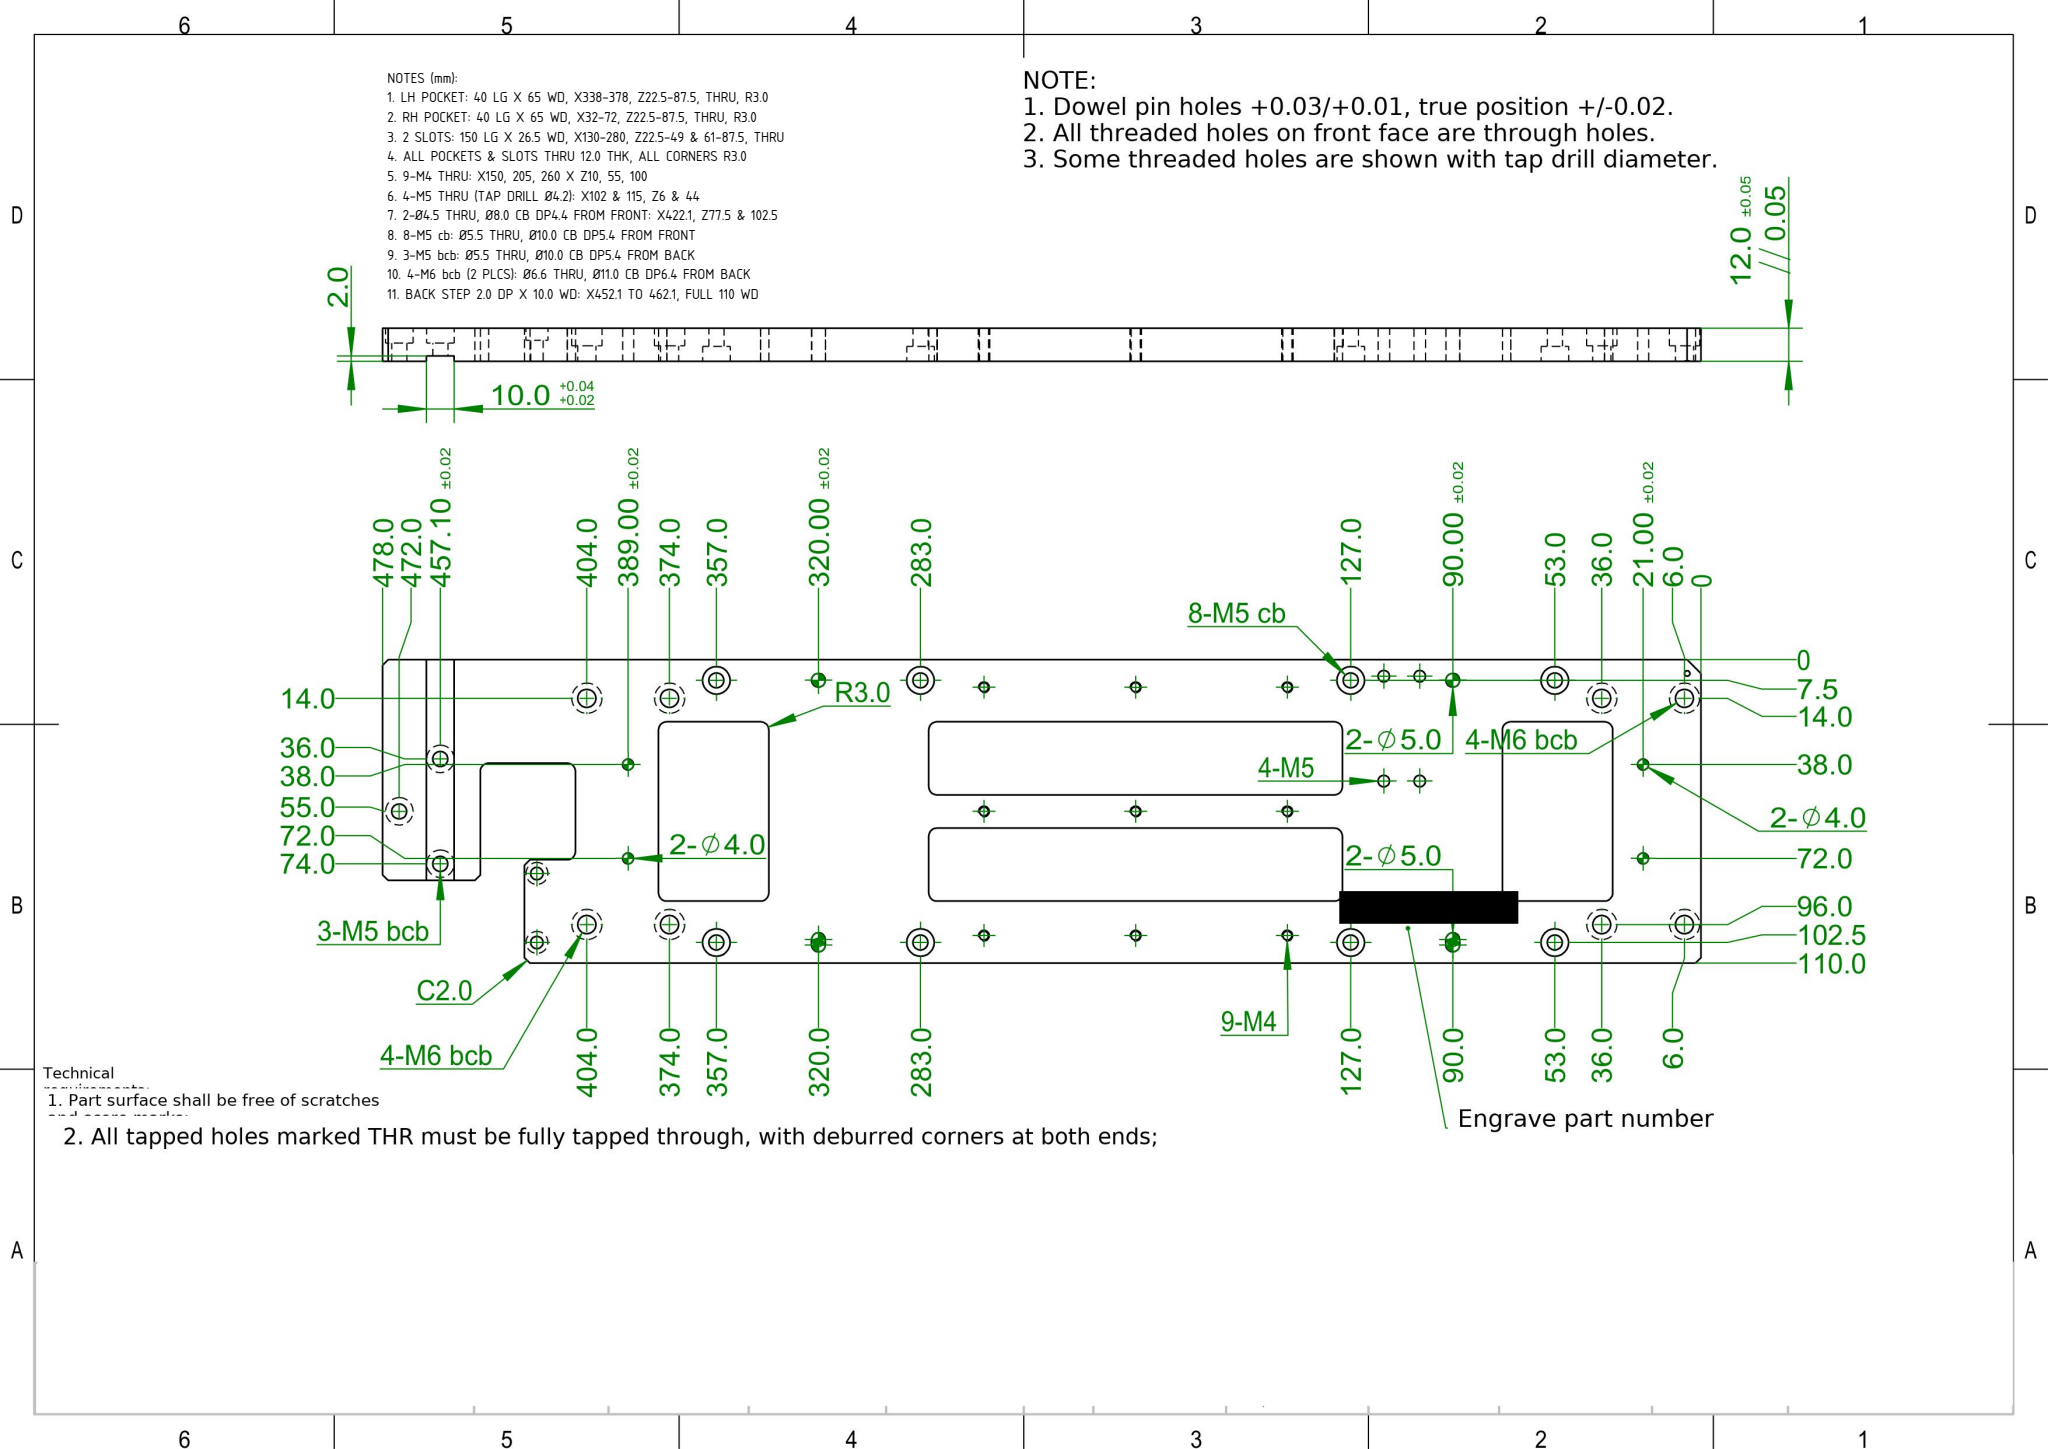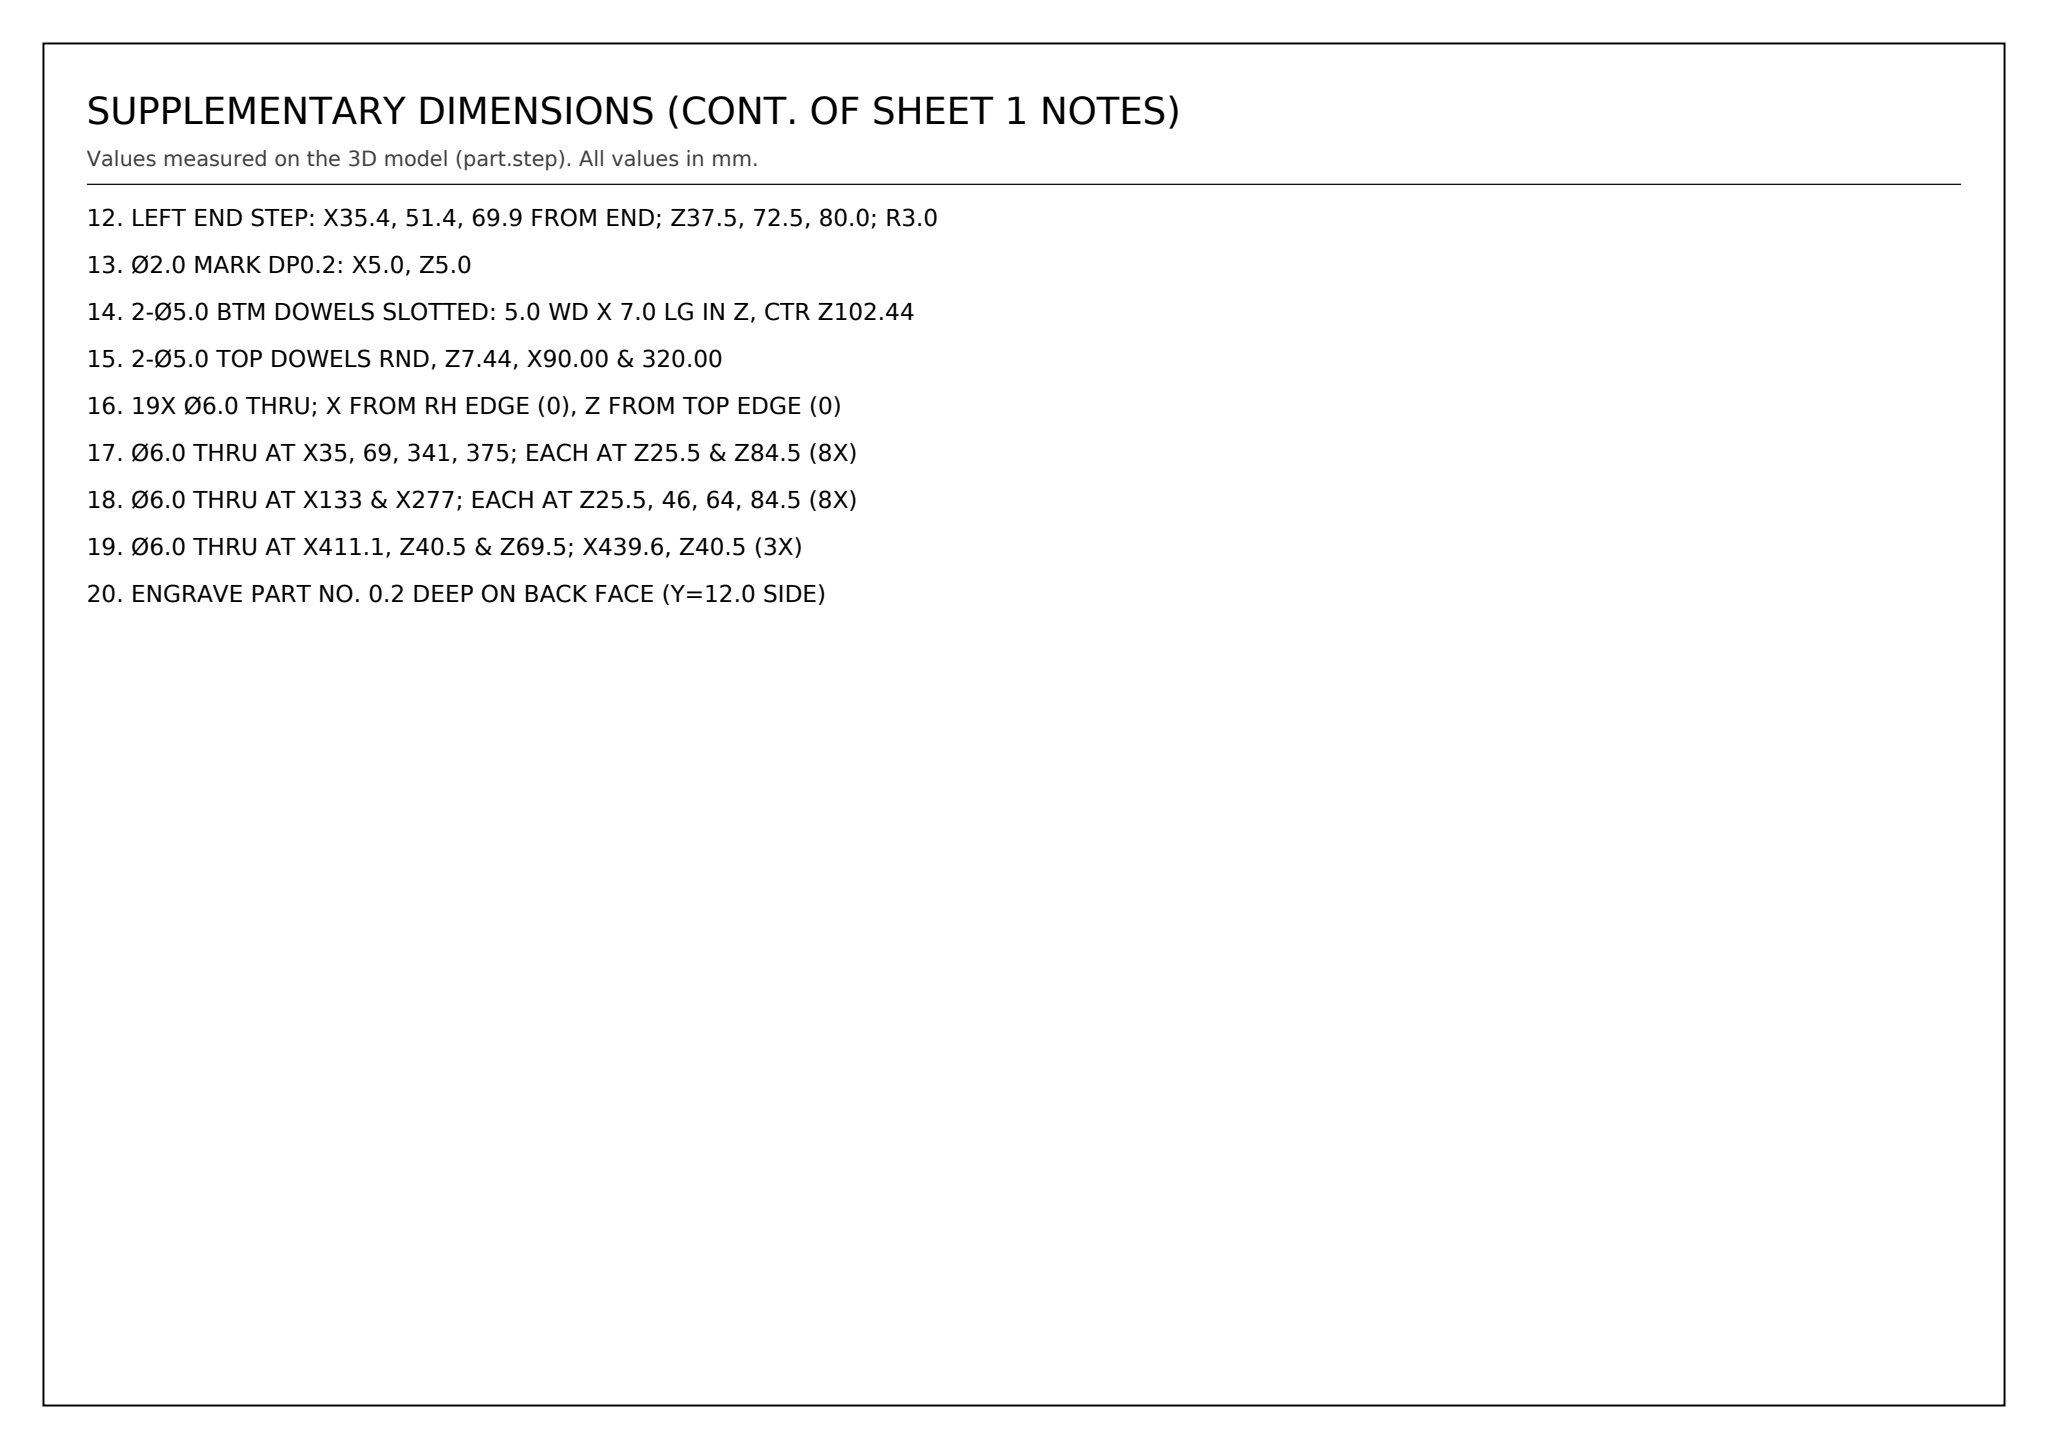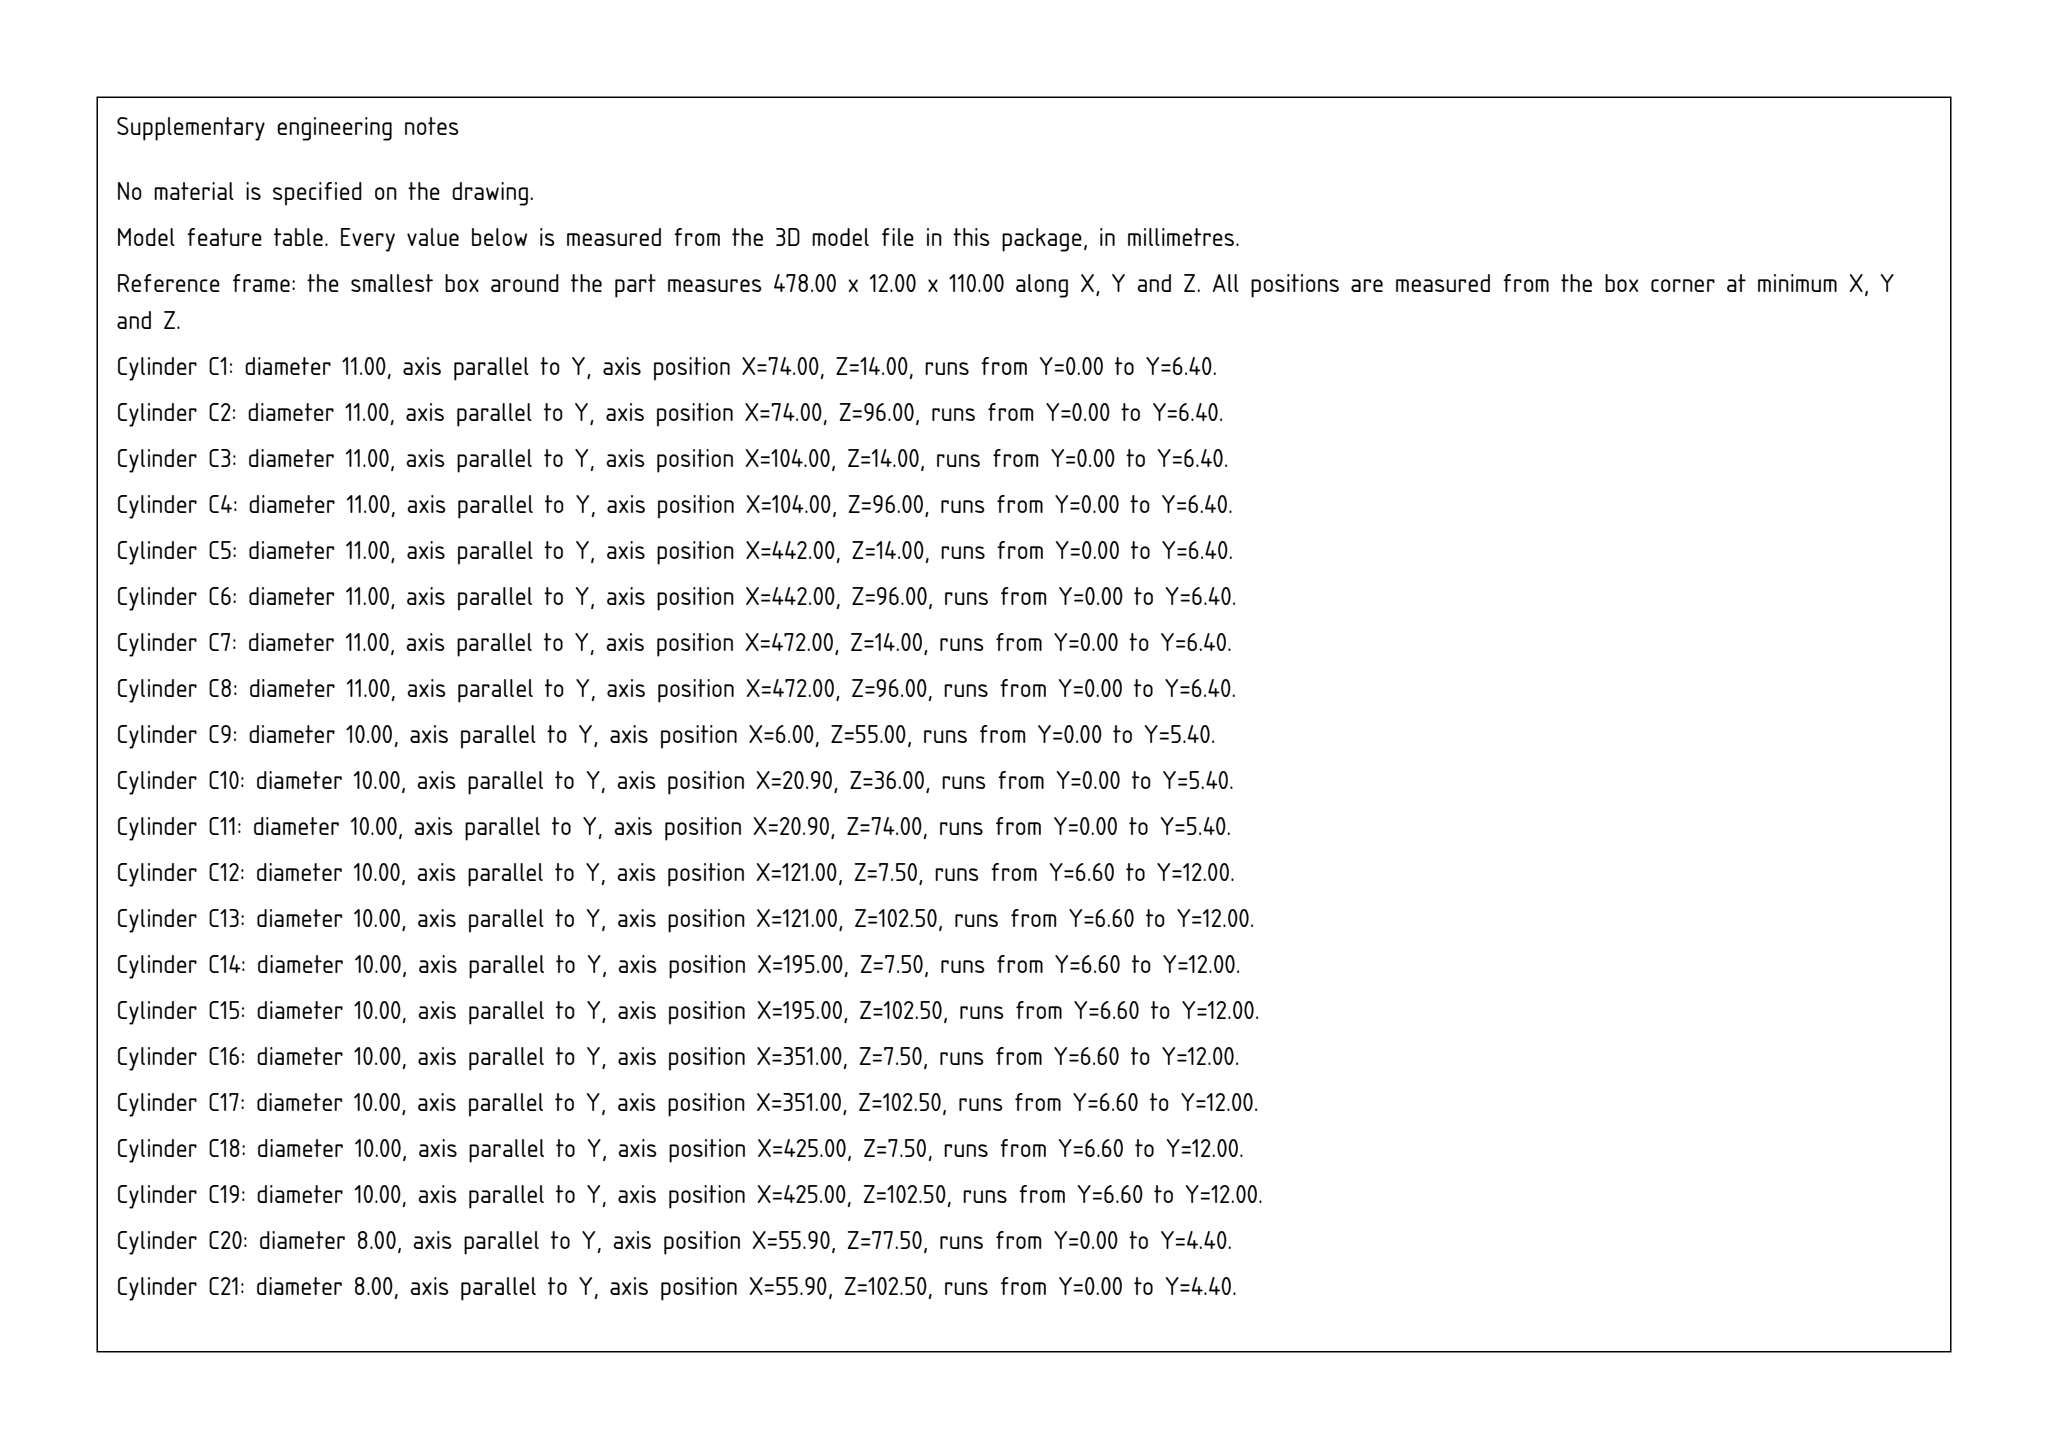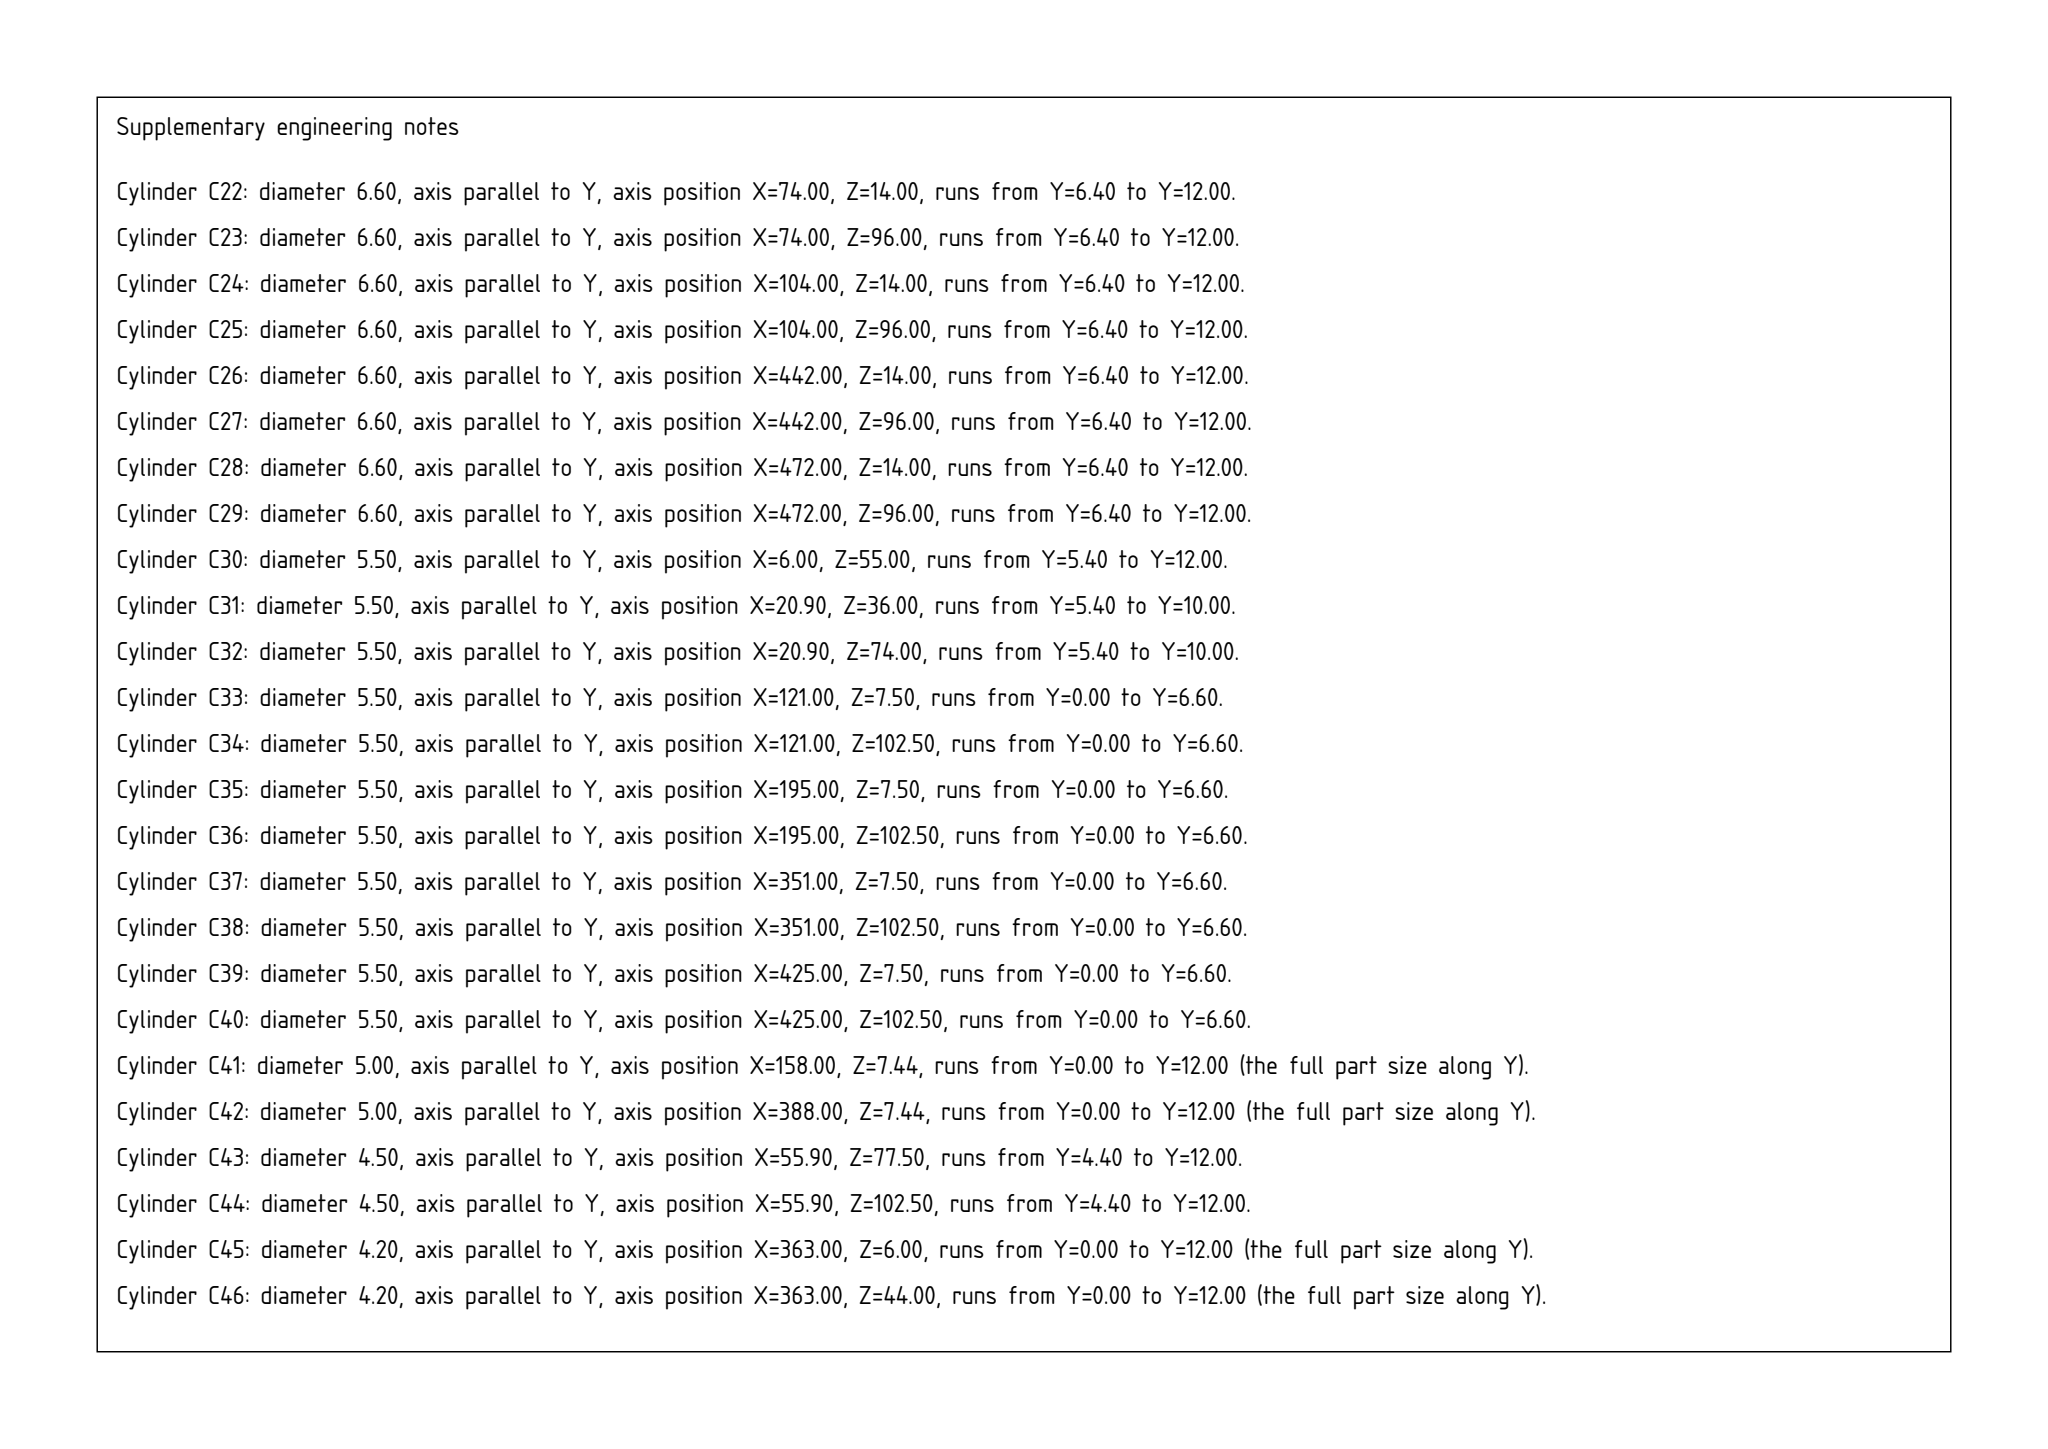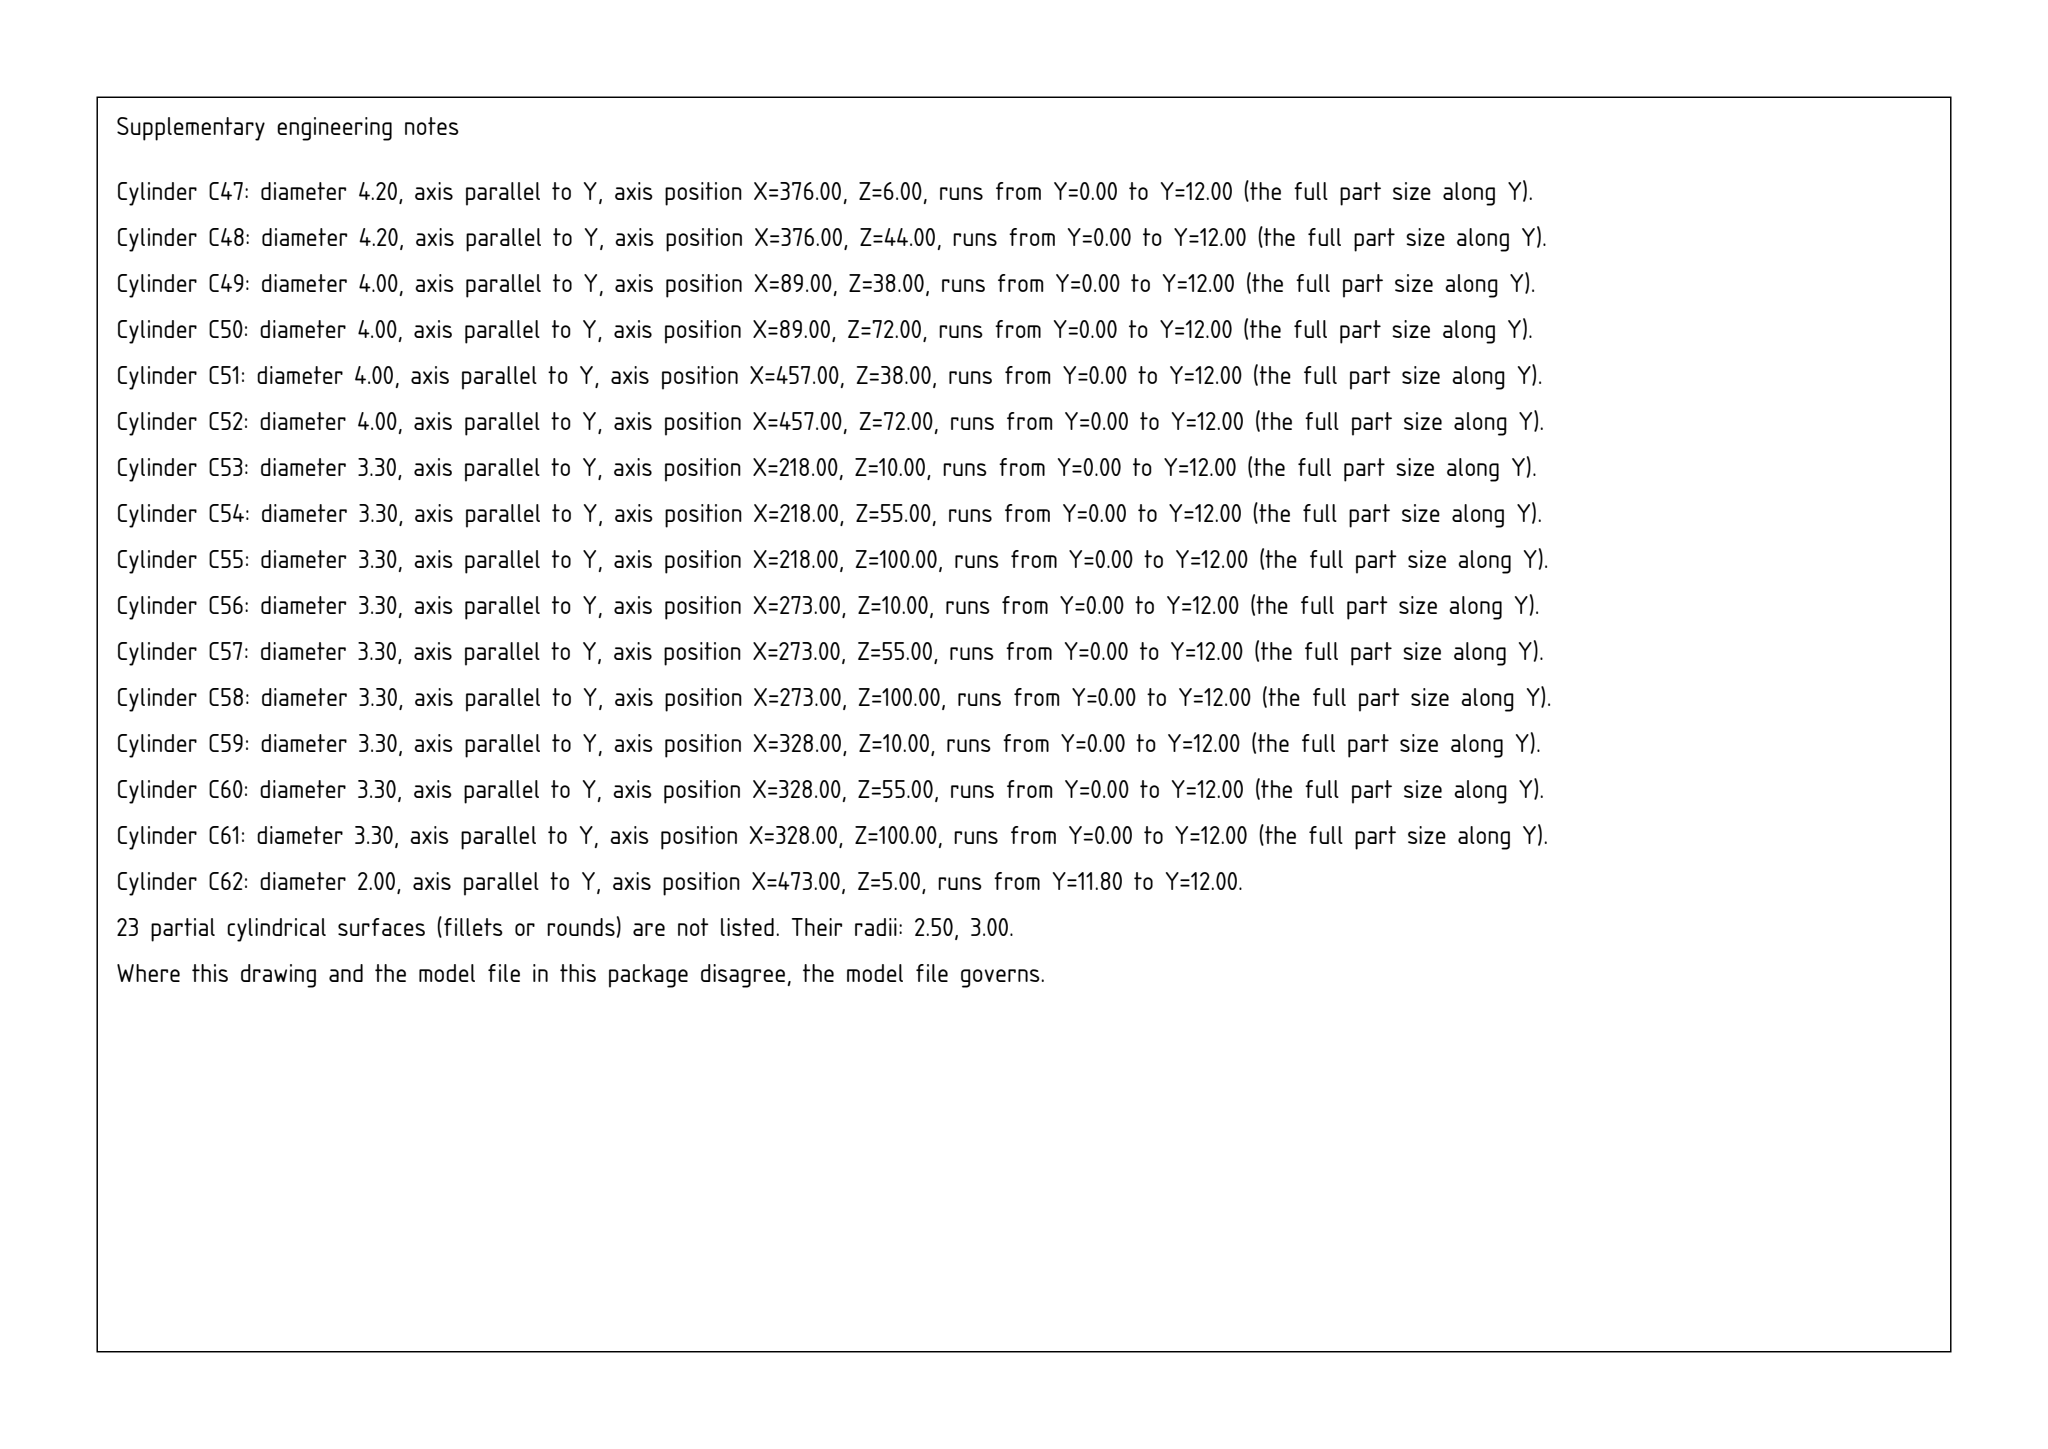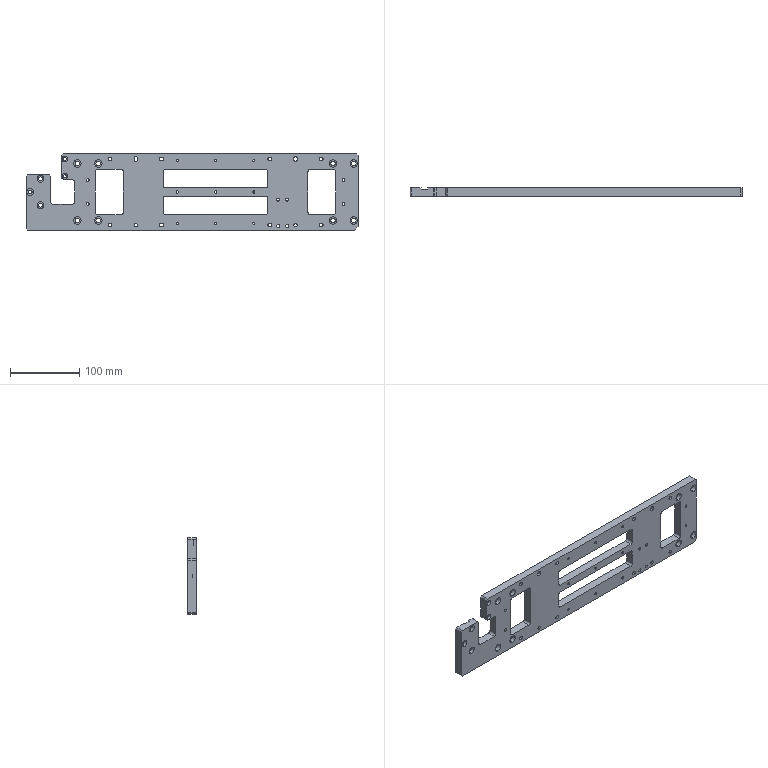Part | SolidWorks | mm | 1 solid | 214 faces | box 478 x 12 x 110 mm | volume 420520 mm3 | cylinder 149 | plane 65 | commonest cylinder face diameters 10 x22 5.5 x22 6 x19 3.3 x18 11 x16 6.6 x16 5 x10 4 x8
Drawing notes:
LH POCKET: 40 LG X 65 WD, X338-378, Z22.5-87.5, THRU, R3.0 | from the solid: x planes 100/140, z planes 22.5/87.5, R3 corner cyls dia6 len12 (thru 12)
RH POCKET: 40 LG X 65 WD, X32-72, Z22.5-87.5, THRU, R3.0 | from the solid: x planes 406/446, z 22.5/87.5, corner cyls dia6 at x409/443, z25.5/84.5, len12
2 SLOTS: 150 LG X 26.5 WD, X130-280, Z22.5-49 & 61-87.5, THRU | from the solid: x planes 198/348, z planes 22.5/49/61/87.5, corner cyls dia6 len12 at x201/345
ALL POCKETS & SLOTS THRU 12.0 THK, ALL CORNERS R3.0 | from the solid: corner cylinders length 12.0 = bbox y thickness 12.0
9-M4 THRU: X150, 205, 260 X Z10, 55, 100 | from the solid: dia3.3 y-holes len12 at x218/273/328 (=478-X), z10/55/100
4-M5 THRU (TAP DRILL Ø4.2): X102 & 115, Z6 & 44 | from the solid: dia4.2 y-holes len12 at x363/376, z6/44
2-Ø4.5 THRU, Ø8.0 CB DP4.4 FROM FRONT: X422.1, Z77.5 & 102.5 | from the solid: dia4.5 len7.6 + dia8.0 len4.4 at x55.9, z77.5 & 102.5
8-M5 cb: Ø5.5 THRU, Ø10.0 CB DP5.4 FROM FRONT | from the solid: dia5.5 len6.6 + dia10.0 len5.4 at x121/195/351/425, z7.5/102.5
3-M5 bcb: Ø5.5 THRU, Ø10.0 CB DP5.4 FROM BACK | from the solid: dia5.5 (6.6/4.6 len) + dia10.0 len5.4 at x6 z55, x20.9 z36 & 74
4-M6 bcb (2 PLCS): Ø6.6 THRU, Ø11.0 CB DP6.4 FROM BACK | from the solid: dia6.6 len5.6 + dia11.0 len6.4 at x74/104/442/472, z14/96
BACK STEP 2.0 DP X 10.0 WD: X452.1 TO 462.1, FULL 110 WD | from the solid: x planes 15.9/25.9 (=478-452.1/-462.1), y plane 10.0 vs 12.0 thk
LEFT END STEP: X35.4, 51.4, 69.9 FROM END; Z37.5, 72.5, 80.0; R3.0 | from the solid: x planes 35.4/51.4/69.9, z planes 37.5/72.5/80.0, dia6 corner cyls at (38.4,40.5),(66.9,40.5),(66.9,69.5)
Ø2.0 MARK DP0.2: X5.0, Z5.0 | from the solid: dia2.0 y-cyl len0.2 at x473 (=478-5.0), z5.0
2-Ø5.0 BTM DOWELS SLOTTED: 5.0 WD X 7.0 LG IN Z, CTR Z102.44 | from the solid: dia5.0 len12 end ctrs z101.44 & 103.44 at x158 & 388
2-Ø5.0 TOP DOWELS RND, Z7.44, X90.00 & 320.00 | from the solid: dia5.0 len12 at x158/388, z7.44
19X Ø6.0 THRU; X FROM RH EDGE (0), Z FROM TOP EDGE (0) | from the solid: 19 cylinders dia 6.0, axis Y, length 12.0 = full 12.0 plate thk; drawing X = 478 - x_step, Z = z_step
Ø6.0 THRU AT X35, 69, 341, 375; EACH AT Z25.5 & Z84.5 (8X) | from the solid: dia6.0 at x443,409,137,103 (=478-x: 35,69,341,375) with z 25.5 and 84.5
Ø6.0 THRU AT X133 & X277; EACH AT Z25.5, 46, 64, 84.5 (8X) | from the solid: dia6.0 at x345 and x201 (=478-x: 133, 277), z 25.5, 46.0, 64.0, 84.5
Ø6.0 THRU AT X411.1, Z40.5 & Z69.5; X439.6, Z40.5 (3X) | from the solid: dia6.0 at x66.9 z40.5/69.5 and x38.4 z40.5 (=478-x: 411.1, 439.6)
ENGRAVE PART NO. 0.2 DEEP ON BACK FACE (Y=12.0 SIDE) | from the solid: dia2.0 y-axis mark, length 0.2, and y plane at 11.8 vs 12.0 back face